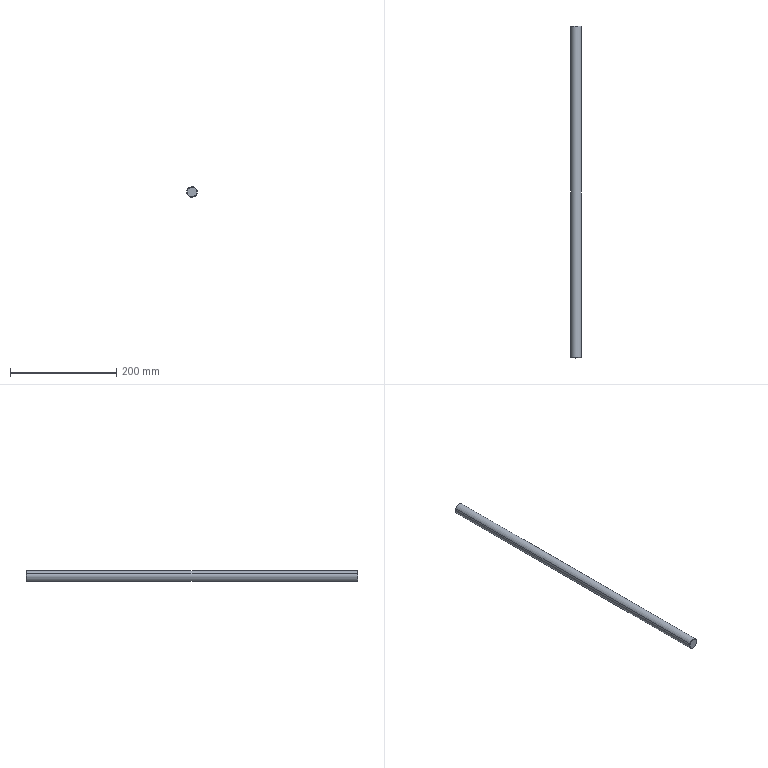Component | SolidWorks | YC1-250-04BalancerAssembly#16673-1_YC1-250-04-10Double-endedScrew#16673-1 | 1 solid | 8 faces | box 20 x 625 x 20 mm | volume 196289 mm3 | cone 4 | cylinder 2 | plane 2 | commonest cylinder face diameters 20 x2 | material Plain Carbon Steel
STEP:
#1=COLOUR_RGB('',0.7922,0.8196,0.9333);
#2=FILL_AREA_STYLE_COLOUR('',#1);
#3=FILL_AREA_STYLE('',(#2));
#4=SURFACE_STYLE_FILL_AREA(#3);
#5=SURFACE_SIDE_STYLE('',(#4));
#6=SURFACE_STYLE_USAGE(.BOTH.,#5);
#7=PRESENTATION_STYLE_ASSIGNMENT((#6));
#8=CARTESIAN_POINT('',(-13.731,161.654,-4.56));
#9=VERTEX_POINT('',#8);
#10=CARTESIAN_POINT('',(-13.024,161.654,-4.906));
#11=VERTEX_POINT('',#10);
#12=CARTESIAN_POINT('',(-13.378,161.654,-4.733));
#13=DIRECTION('',(-0.,1.,0.));
#14=DIRECTION('',(-0.8982,0.,0.4395));
#15=AXIS2_PLACEMENT_3D('',#12,#13,#14);
#16=CIRCLE('',#15,0.3937);
#17=EDGE_CURVE('',#9,#11,#16,.T.);
#18=ORIENTED_EDGE('',*,*,#17,.T.);
#19=CARTESIAN_POINT('',(-13.024,186.181,-4.906));
#20=VERTEX_POINT('',#19);
#21=CARTESIAN_POINT('',(-13.024,161.614,-4.906));
#22=DIRECTION('',(-0.,1.,0.));
#23=VECTOR('',#22,39.37);
#24=LINE('',#21,#23);
#25=EDGE_CURVE('',#11,#20,#24,.T.);
#26=ORIENTED_EDGE('',*,*,#25,.T.);
#27=CARTESIAN_POINT('',(-13.731,186.181,-4.56));
#28=VERTEX_POINT('',#27);
#29=CARTESIAN_POINT('',(-13.378,186.181,-4.733));
#30=DIRECTION('',(0.,-1.,-0.));
#31=DIRECTION('',(-0.8982,0.,0.4395));
#32=AXIS2_PLACEMENT_3D('',#29,#30,#31);
#33=CIRCLE('',#32,0.3937);
#34=EDGE_CURVE('',#20,#28,#33,.T.);
#35=ORIENTED_EDGE('',*,*,#34,.T.);
#36=CARTESIAN_POINT('',(-13.731,161.614,-4.56));
#37=DIRECTION('',(-0.,1.,0.));
#38=VECTOR('',#37,39.37);
#39=LINE('',#36,#38);
#40=EDGE_CURVE('',#9,#28,#39,.T.);
#41=ORIENTED_EDGE('',*,*,#40,.F.);
#42=EDGE_LOOP('',(#18,#26,#35,#41));
#43=FACE_OUTER_BOUND('',#42,.T.);
#44=CARTESIAN_POINT('',(-13.378,161.614,-4.733));
#45=DIRECTION('',(-0.,1.,0.));
#46=DIRECTION('',(-0.8982,0.,0.4395));
#47=AXIS2_PLACEMENT_3D('',#44,#45,#46);
#48=CYLINDRICAL_SURFACE('',#47,0.3937);
#49=ADVANCED_FACE('',(#43),#48,.T.);
#50=CARTESIAN_POINT('',(-13.059,186.22,-4.888));
#51=VERTEX_POINT('',#50);
#52=CARTESIAN_POINT('',(-13.696,186.22,-4.577));
#53=VERTEX_POINT('',#52);
#54=CARTESIAN_POINT('',(-13.378,186.22,-4.733));
#55=DIRECTION('',(0.,-1.,-0.));
#56=DIRECTION('',(0.8982,0.,-0.4395));
#57=AXIS2_PLACEMENT_3D('',#54,#55,#56);
#58=CIRCLE('',#57,0.3543);
#59=EDGE_CURVE('',#51,#53,#58,.T.);
#60=ORIENTED_EDGE('',*,*,#59,.T.);
#61=CARTESIAN_POINT('',(-13.731,186.181,-4.56));
#62=DIRECTION('',(-0.6352,-0.7071,0.3108));
#63=VECTOR('',#62,39.37);
#64=LINE('',#61,#63);
#65=EDGE_CURVE('',#53,#28,#64,.T.);
#66=ORIENTED_EDGE('',*,*,#65,.T.);
#67=ORIENTED_EDGE('',*,*,#34,.F.);
#68=CARTESIAN_POINT('',(-13.024,186.181,-4.906));
#69=DIRECTION('',(0.6352,-0.7071,-0.3108));
#70=VECTOR('',#69,39.37);
#71=LINE('',#68,#70);
#72=EDGE_CURVE('',#51,#20,#71,.T.);
#73=ORIENTED_EDGE('',*,*,#72,.F.);
#74=EDGE_LOOP('',(#60,#66,#67,#73));
#75=FACE_OUTER_BOUND('',#74,.T.);
#76=CARTESIAN_POINT('',(-13.378,186.181,-4.733));
#77=DIRECTION('',(0.,-1.,-0.));
#78=DIRECTION('',(0.8982,0.,-0.4395));
#79=AXIS2_PLACEMENT_3D('',#76,#77,#78);
#80=CONICAL_SURFACE('',#79,0.3937,0.7854);
#81=ADVANCED_FACE('',(#75),#80,.T.);
#82=CARTESIAN_POINT('',(-13.696,161.614,-4.577));
#83=VERTEX_POINT('',#82);
#84=CARTESIAN_POINT('',(-13.059,161.614,-4.888));
#85=VERTEX_POINT('',#84);
#86=CARTESIAN_POINT('',(-13.378,161.614,-4.733));
#87=DIRECTION('',(-0.,1.,0.));
#88=DIRECTION('',(-0.8982,0.,0.4395));
#89=AXIS2_PLACEMENT_3D('',#86,#87,#88);
#90=CIRCLE('',#89,0.3543);
#91=EDGE_CURVE('',#83,#85,#90,.T.);
#92=ORIENTED_EDGE('',*,*,#91,.T.);
#93=CARTESIAN_POINT('',(-13.024,161.654,-4.906));
#94=DIRECTION('',(0.6352,0.7071,-0.3108));
#95=VECTOR('',#94,39.37);
#96=LINE('',#93,#95);
#97=EDGE_CURVE('',#85,#11,#96,.T.);
#98=ORIENTED_EDGE('',*,*,#97,.T.);
#99=ORIENTED_EDGE('',*,*,#17,.F.);
#100=CARTESIAN_POINT('',(-13.731,161.654,-4.56));
#101=DIRECTION('',(-0.6352,0.7071,0.3108));
#102=VECTOR('',#101,39.37);
#103=LINE('',#100,#102);
#104=EDGE_CURVE('',#83,#9,#103,.T.);
#105=ORIENTED_EDGE('',*,*,#104,.F.);
#106=EDGE_LOOP('',(#92,#98,#99,#105));
#107=FACE_OUTER_BOUND('',#106,.T.);
#108=CARTESIAN_POINT('',(-13.378,161.654,-4.733));
#109=DIRECTION('',(-0.,1.,0.));
#110=DIRECTION('',(-0.8982,0.,0.4395));
#111=AXIS2_PLACEMENT_3D('',#108,#109,#110);
#112=CONICAL_SURFACE('',#111,0.3937,0.7854);
#113=ADVANCED_FACE('',(#107),#112,.T.);
#114=ORIENTED_EDGE('',*,*,#25,.F.);
#115=CARTESIAN_POINT('',(-13.378,161.654,-4.733));
#116=DIRECTION('',(-0.,1.,0.));
#117=DIRECTION('',(-0.8982,0.,0.4395));
#118=AXIS2_PLACEMENT_3D('',#115,#116,#117);
#119=CIRCLE('',#118,0.3937);
#120=EDGE_CURVE('',#11,#9,#119,.T.);
#121=ORIENTED_EDGE('',*,*,#120,.T.);
#122=ORIENTED_EDGE('',*,*,#40,.T.);
#123=CARTESIAN_POINT('',(-13.378,186.181,-4.733));
#124=DIRECTION('',(0.,-1.,-0.));
#125=DIRECTION('',(-0.8982,0.,0.4395));
#126=AXIS2_PLACEMENT_3D('',#123,#124,#125);
#127=CIRCLE('',#126,0.3937);
#128=EDGE_CURVE('',#28,#20,#127,.T.);
#129=ORIENTED_EDGE('',*,*,#128,.T.);
#130=EDGE_LOOP('',(#114,#121,#122,#129));
#131=FACE_OUTER_BOUND('',#130,.T.);
#132=CARTESIAN_POINT('',(-13.378,161.614,-4.733));
#133=DIRECTION('',(-0.,1.,0.));
#134=DIRECTION('',(-0.8982,0.,0.4395));
#135=AXIS2_PLACEMENT_3D('',#132,#133,#134);
#136=CYLINDRICAL_SURFACE('',#135,0.3937);
#137=ADVANCED_FACE('',(#131),#136,.T.);
#138=ORIENTED_EDGE('',*,*,#65,.F.);
#139=CARTESIAN_POINT('',(-13.378,186.22,-4.733));
#140=DIRECTION('',(0.,-1.,-0.));
#141=DIRECTION('',(0.8982,0.,-0.4395));
#142=AXIS2_PLACEMENT_3D('',#139,#140,#141);
#143=CIRCLE('',#142,0.3543);
#144=EDGE_CURVE('',#53,#51,#143,.T.);
#145=ORIENTED_EDGE('',*,*,#144,.T.);
#146=ORIENTED_EDGE('',*,*,#72,.T.);
#147=ORIENTED_EDGE('',*,*,#128,.F.);
#148=EDGE_LOOP('',(#138,#145,#146,#147));
#149=FACE_OUTER_BOUND('',#148,.T.);
#150=CARTESIAN_POINT('',(-13.378,186.181,-4.733));
#151=DIRECTION('',(0.,-1.,-0.));
#152=DIRECTION('',(0.8982,0.,-0.4395));
#153=AXIS2_PLACEMENT_3D('',#150,#151,#152);
#154=CONICAL_SURFACE('',#153,0.3937,0.7854);
#155=ADVANCED_FACE('',(#149),#154,.T.);
#156=ORIENTED_EDGE('',*,*,#97,.F.);
#157=CARTESIAN_POINT('',(-13.378,161.614,-4.733));
#158=DIRECTION('',(-0.,1.,0.));
#159=DIRECTION('',(-0.8982,0.,0.4395));
#160=AXIS2_PLACEMENT_3D('',#157,#158,#159);
#161=CIRCLE('',#160,0.3543);
#162=EDGE_CURVE('',#85,#83,#161,.T.);
#163=ORIENTED_EDGE('',*,*,#162,.T.);
#164=ORIENTED_EDGE('',*,*,#104,.T.);
#165=ORIENTED_EDGE('',*,*,#120,.F.);
#166=EDGE_LOOP('',(#156,#163,#164,#165));
#167=FACE_OUTER_BOUND('',#166,.T.);
#168=CARTESIAN_POINT('',(-13.378,161.654,-4.733));
#169=DIRECTION('',(-0.,1.,0.));
#170=DIRECTION('',(-0.8982,0.,0.4395));
#171=AXIS2_PLACEMENT_3D('',#168,#169,#170);
#172=CONICAL_SURFACE('',#171,0.3937,0.7854);
#173=ADVANCED_FACE('',(#167),#172,.T.);
#174=ORIENTED_EDGE('',*,*,#59,.F.);
#175=ORIENTED_EDGE('',*,*,#144,.F.);
#176=EDGE_LOOP('',(#174,#175));
#177=FACE_OUTER_BOUND('',#176,.T.);
#178=CARTESIAN_POINT('',(-13.378,186.22,-4.733));
#179=DIRECTION('',(0.,-1.,-0.));
#180=DIRECTION('',(0.8982,0.,-0.4395));
#181=AXIS2_PLACEMENT_3D('',#178,#179,#180);
#182=PLANE('',#181);
#183=ADVANCED_FACE('',(#177),#182,.F.);
#184=ORIENTED_EDGE('',*,*,#91,.F.);
#185=ORIENTED_EDGE('',*,*,#162,.F.);
#186=EDGE_LOOP('',(#184,#185));
#187=FACE_OUTER_BOUND('',#186,.T.);
#188=CARTESIAN_POINT('',(-13.378,161.614,-4.733));
#189=DIRECTION('',(0.,-1.,-0.));
#190=DIRECTION('',(0.8982,0.,-0.4395));
#191=AXIS2_PLACEMENT_3D('',#188,#189,#190);
#192=PLANE('',#191);
#193=ADVANCED_FACE('',(#187),#192,.T.);
#194=CLOSED_SHELL('',(#49,#81,#113,#137,#155,#173,#183,#193));
#195=MANIFOLD_SOLID_BREP('',#194);
#196=STYLED_ITEM('',(#7),#195);
#197=PRESENTATION_LAYER_ASSIGNMENT('','',(#196));
#198=CARTESIAN_POINT('',(0.,0.,0.));
#199=DIRECTION('',(0.,0.,1.));
#200=DIRECTION('',(1.,0.,0.));
#201=AXIS2_PLACEMENT_3D('',#198,#199,#200);
#202=(LENGTH_UNIT()NAMED_UNIT(*)SI_UNIT($,.METRE.));
#203=LENGTH_MEASURE_WITH_UNIT(LENGTH_MEASURE(0.0254),#202);
#204=DIMENSIONAL_EXPONENTS(1.,0.,0.,0.,0.,0.,0.);
#205=(CONVERSION_BASED_UNIT('',#203)LENGTH_UNIT()NAMED_UNIT(#204));
#206=UNCERTAINTY_MEASURE_WITH_UNIT(LENGTH_MEASURE(0.00001),#205,'','');
#207=(NAMED_UNIT(*)PLANE_ANGLE_UNIT()SI_UNIT($,.RADIAN.));
#208=(NAMED_UNIT(*)SI_UNIT($,.STERADIAN.)SOLID_ANGLE_UNIT());
#209=(GEOMETRIC_REPRESENTATION_CONTEXT(3)GLOBAL_UNCERTAINTY_ASSIGNED_CONTEXT((#206))GLOBAL_UNIT_ASSIGNED_CONTEXT((#205,#207,#208))REPRESENTATION_CONTEXT('',''));
#210=ADVANCED_BREP_SHAPE_REPRESENTATION('',(#195,#201),#209);
#211=(LENGTH_UNIT()NAMED_UNIT(*)SI_UNIT($,.METRE.));
#212=LENGTH_MEASURE_WITH_UNIT(LENGTH_MEASURE(0.0254),#211);
#213=DIMENSIONAL_EXPONENTS(1.,0.,0.,0.,0.,0.,0.);
#214=(CONVERSION_BASED_UNIT('',#212)LENGTH_UNIT()NAMED_UNIT(#213));
#215=UNCERTAINTY_MEASURE_WITH_UNIT(LENGTH_MEASURE(0.00001),#214,'','');
#216=(NAMED_UNIT(*)PLANE_ANGLE_UNIT()SI_UNIT($,.RADIAN.));
#217=(NAMED_UNIT(*)SI_UNIT($,.STERADIAN.)SOLID_ANGLE_UNIT());
#218=(GEOMETRIC_REPRESENTATION_CONTEXT(3)GLOBAL_UNCERTAINTY_ASSIGNED_CONTEXT((#215))GLOBAL_UNIT_ASSIGNED_CONTEXT((#214,#216,#217))REPRESENTATION_CONTEXT('',''));
#219=MECHANICAL_DESIGN_GEOMETRIC_PRESENTATION_REPRESENTATION('',(#196),#218);